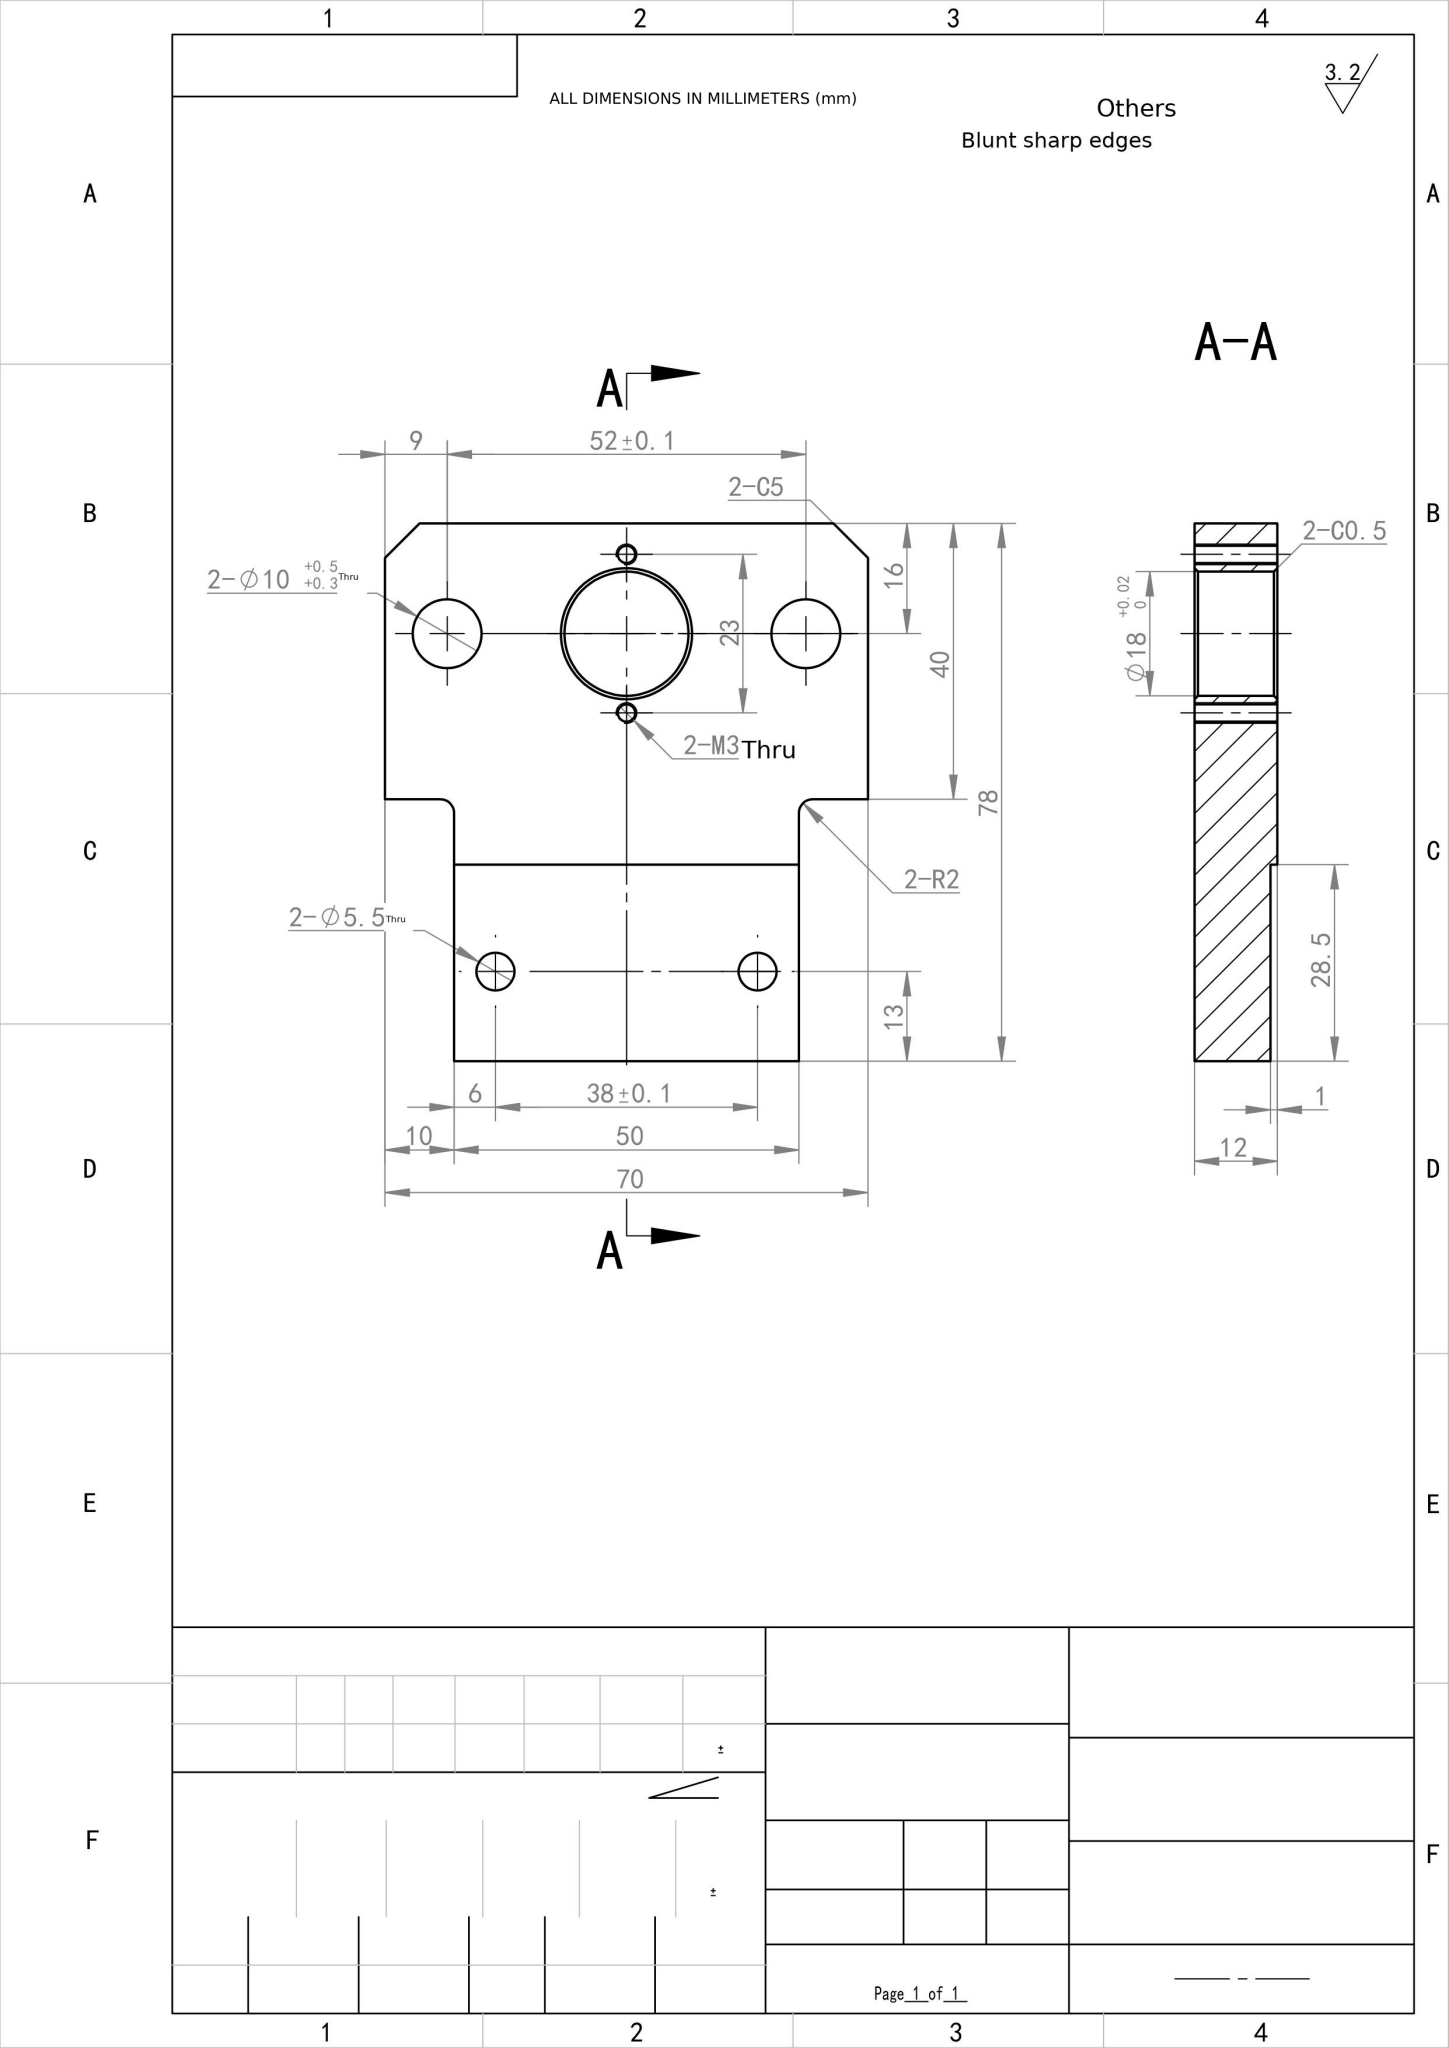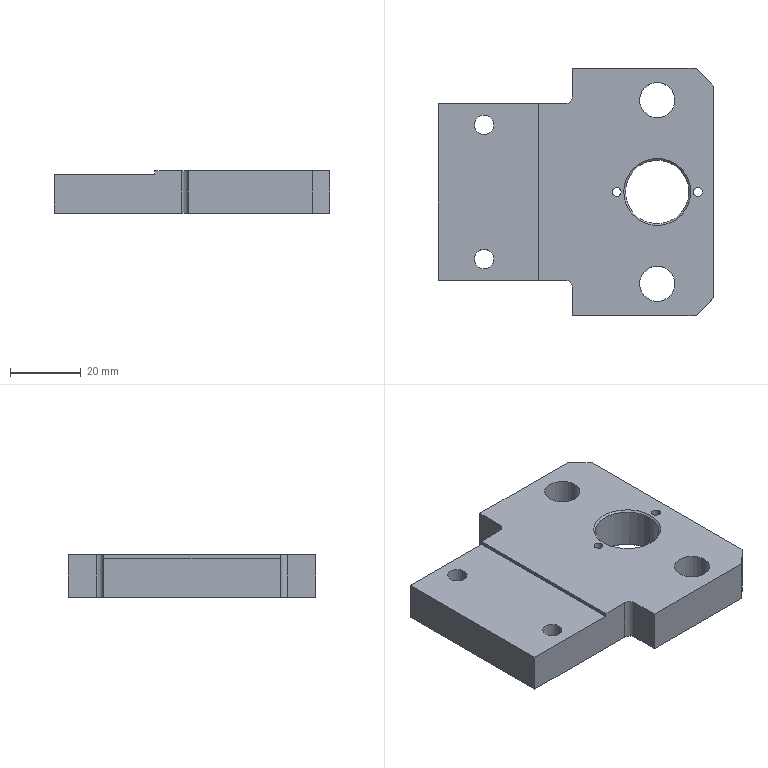Part | NX | mm | 1 solid | 34 faces | box 78 x 70 x 12 mm | volume 49102 mm3 | cylinder 16 | plane 14 | cone 4 | commonest cylinder face diameters 2.5 x4 5.5 x4 10 x4 18 x2 4 x2